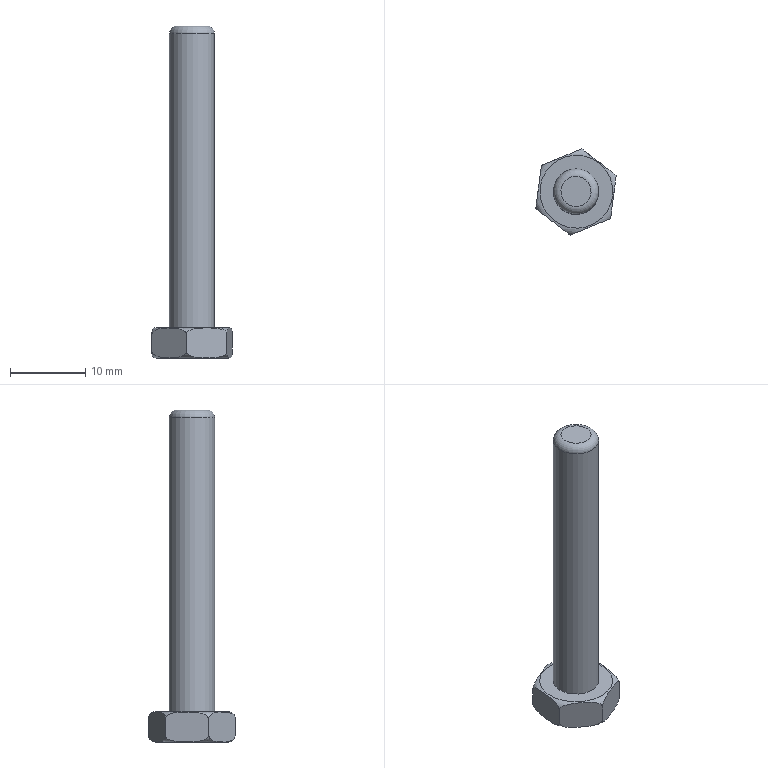Component | NX | BOLT | 1 solid | 13 faces | volume 1472 mm3 | plane 9 | other 2 | cylinder 1 | torus 1 | commonest cylinder face diameters 6 x1